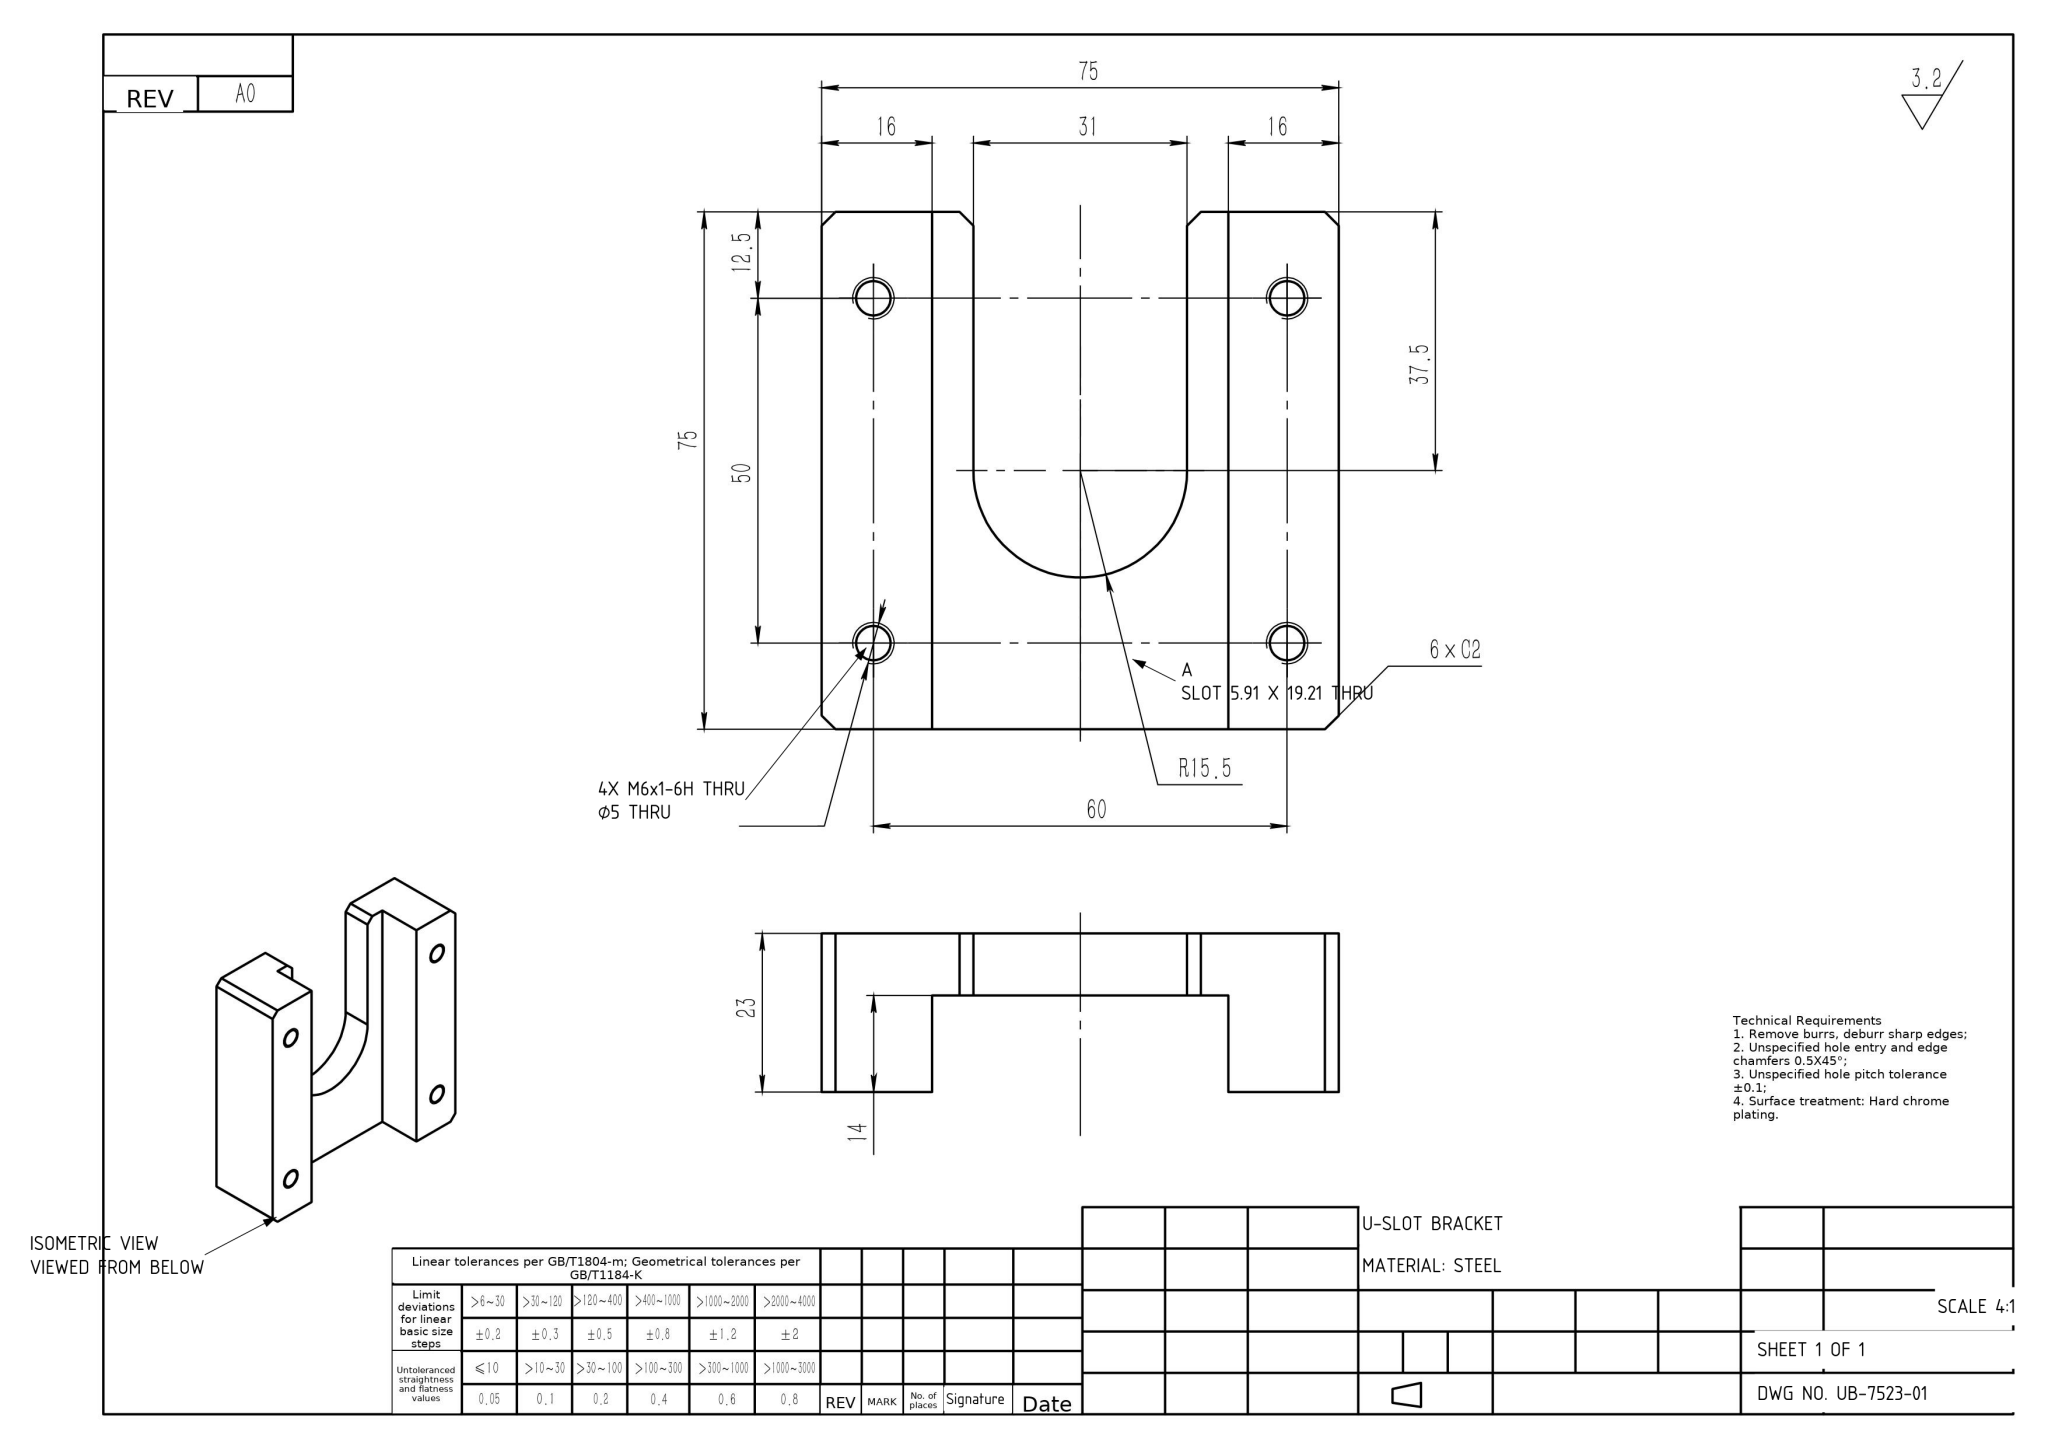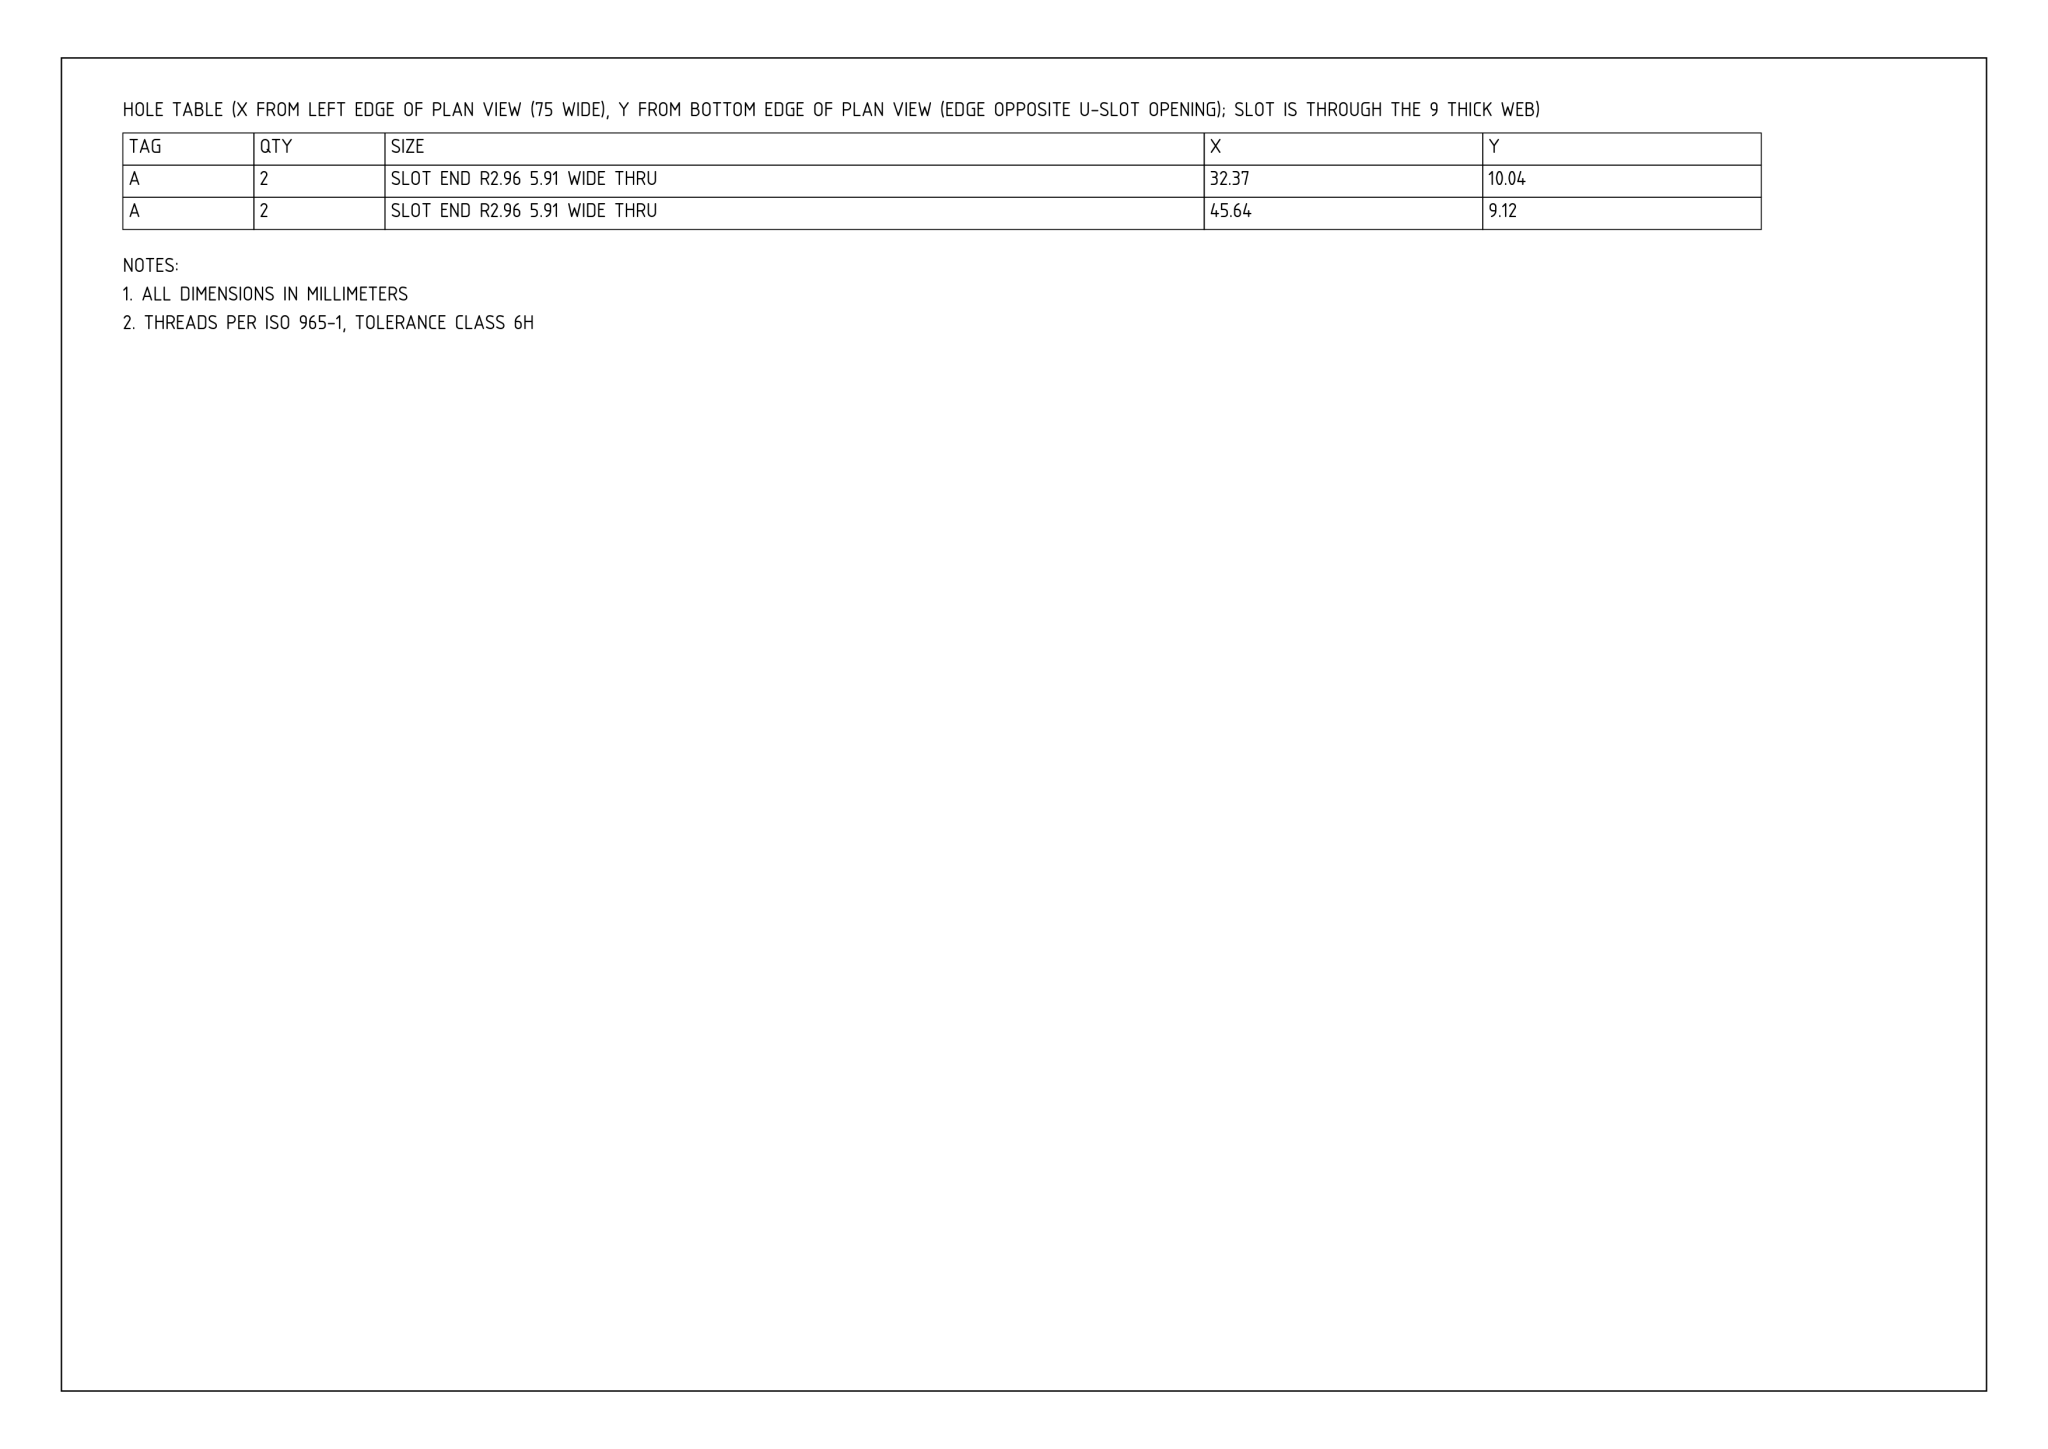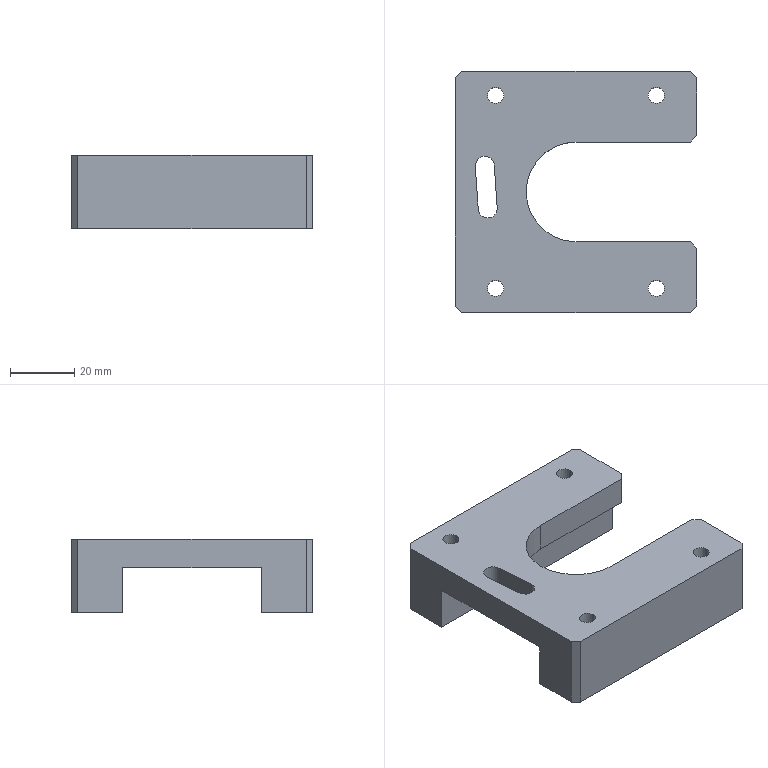Part | NX | mm | 1 solid | 33 faces | box 75 x 75 x 23 mm | volume 67385 mm3 | plane 21 | cylinder 12 | commonest cylinder face diameters 5 x8 5.914 x3 31 x1